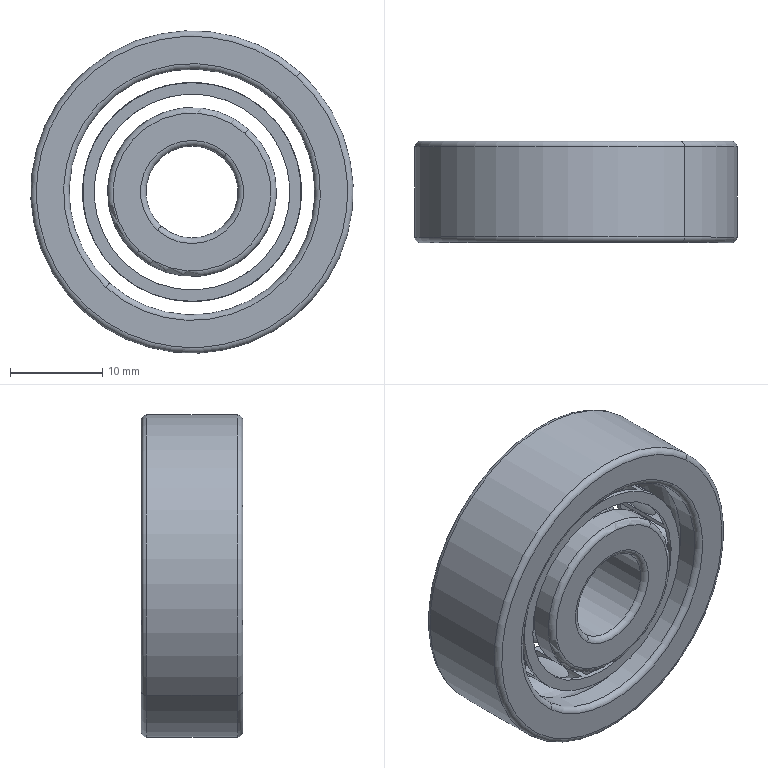Component | SolidWorks | FrontGuideWheel-1_MirrorGuideWheel-3_MirrorGB_T276-2013[DeepGrooveBallBearing[60000]6300]-1 | 12 solids | 119 faces | volume 6277 mm3 | cylinder 55 | plane 24 | torus 22 | sphere 18 | commonest cylinder face diameters 6.975 x19 23.75 x12 21.25 x12 26.667 x4 18.333 x4 35 x2 10 x2 | material AISI 304